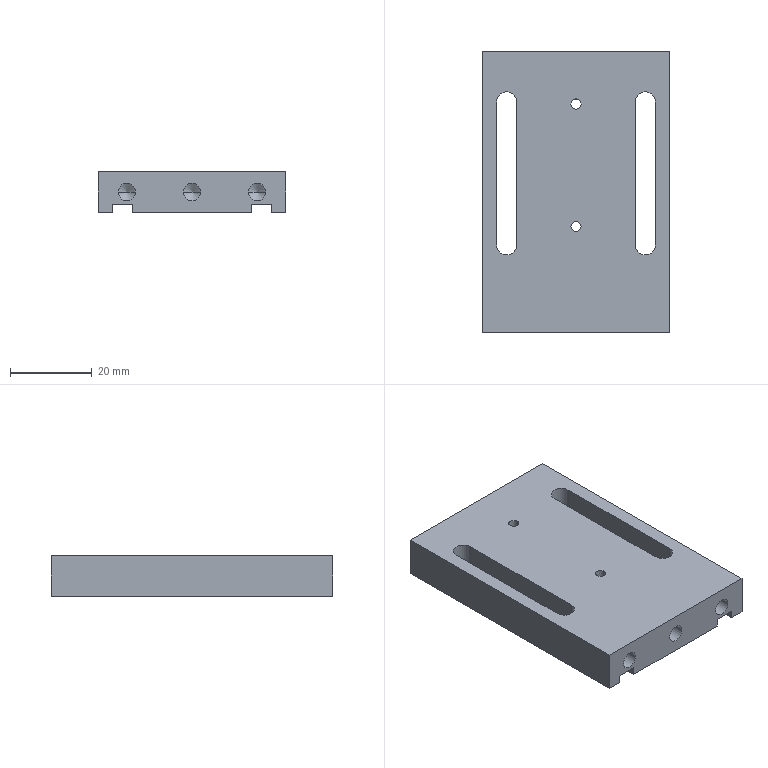Component | SolidWorks | 12-DividingMechanism-1111-1_18-1111-3 | 1 solid | 36 faces | box 46 x 69.1 x 10 mm | volume 26659 mm3 | plane 16 | cylinder 14 | cone 6 | commonest cylinder face diameters 4.2 x6 2.5 x4 5 x4
STEP:
#1=CARTESIAN_POINT('',(0.0523,23.517,60.278));
#2=VERTEX_POINT('',#1);
#3=CARTESIAN_POINT('',(0.2177,23.517,60.278));
#4=VERTEX_POINT('',#3);
#5=CARTESIAN_POINT('',(0.135,23.517,60.278));
#6=DIRECTION('',(-0.,-1.,-0.));
#7=DIRECTION('',(1.,0.,0.));
#8=AXIS2_PLACEMENT_3D('',#5,#6,#7);
#9=CIRCLE('',#8,0.08268);
#10=EDGE_CURVE('',#2,#4,#9,.T.);
#11=ORIENTED_EDGE('',*,*,#10,.F.);
#12=CARTESIAN_POINT('',(0.0523,23.029,60.278));
#13=VERTEX_POINT('',#12);
#14=CARTESIAN_POINT('',(0.0523,23.029,60.278));
#15=DIRECTION('',(-0.,-1.,-0.));
#16=VECTOR('',#15,39.37);
#17=LINE('',#14,#16);
#18=EDGE_CURVE('',#2,#13,#17,.T.);
#19=ORIENTED_EDGE('',*,*,#18,.T.);
#20=CARTESIAN_POINT('',(0.2177,23.029,60.278));
#21=VERTEX_POINT('',#20);
#22=CARTESIAN_POINT('',(0.135,23.029,60.278));
#23=DIRECTION('',(-0.,-1.,-0.));
#24=DIRECTION('',(1.,0.,0.));
#25=AXIS2_PLACEMENT_3D('',#22,#23,#24);
#26=CIRCLE('',#25,0.08268);
#27=EDGE_CURVE('',#13,#21,#26,.T.);
#28=ORIENTED_EDGE('',*,*,#27,.T.);
#29=CARTESIAN_POINT('',(0.2177,23.029,60.278));
#30=DIRECTION('',(-0.,-1.,-0.));
#31=VECTOR('',#30,39.37);
#32=LINE('',#29,#31);
#33=EDGE_CURVE('',#4,#21,#32,.T.);
#34=ORIENTED_EDGE('',*,*,#33,.F.);
#35=EDGE_LOOP('',(#11,#19,#28,#34));
#36=FACE_OUTER_BOUND('',#35,.T.);
#37=CARTESIAN_POINT('',(0.135,23.029,60.278));
#38=DIRECTION('',(-0.,-1.,-0.));
#39=DIRECTION('',(1.,0.,0.));
#40=AXIS2_PLACEMENT_3D('',#37,#38,#39);
#41=CYLINDRICAL_SURFACE('',#40,0.08268);
#42=ADVANCED_FACE('',(#36),#41,.F.);
#43=CARTESIAN_POINT('',(0.135,23.566,60.278));
#44=VERTEX_POINT('',#43);
#45=CARTESIAN_POINT('',(0.2177,23.517,60.278));
#46=DIRECTION('',(0.8572,-0.515,-0.));
#47=VECTOR('',#46,39.37);
#48=LINE('',#45,#47);
#49=EDGE_CURVE('',#44,#4,#48,.T.);
#50=ORIENTED_EDGE('',*,*,#49,.F.);
#51=CARTESIAN_POINT('',(0.0523,23.517,60.278));
#52=DIRECTION('',(-0.8572,-0.515,0.));
#53=VECTOR('',#52,39.37);
#54=LINE('',#51,#53);
#55=EDGE_CURVE('',#44,#2,#54,.T.);
#56=ORIENTED_EDGE('',*,*,#55,.T.);
#57=ORIENTED_EDGE('',*,*,#10,.T.);
#58=EDGE_LOOP('',(#50,#56,#57));
#59=FACE_OUTER_BOUND('',#58,.T.);
#60=CARTESIAN_POINT('',(0.135,23.517,60.278));
#61=DIRECTION('',(-0.,-1.,-0.));
#62=DIRECTION('',(1.,0.,0.));
#63=AXIS2_PLACEMENT_3D('',#60,#61,#62);
#64=CONICAL_SURFACE('',#63,0.08268,1.03);
#65=ADVANCED_FACE('',(#59),#64,.F.);
#66=CARTESIAN_POINT('',(-0.5776,23.517,60.278));
#67=VERTEX_POINT('',#66);
#68=CARTESIAN_POINT('',(-0.4123,23.517,60.278));
#69=VERTEX_POINT('',#68);
#70=CARTESIAN_POINT('',(-0.4949,23.517,60.278));
#71=DIRECTION('',(-0.,-1.,-0.));
#72=DIRECTION('',(1.,0.,0.));
#73=AXIS2_PLACEMENT_3D('',#70,#71,#72);
#74=CIRCLE('',#73,0.08268);
#75=EDGE_CURVE('',#67,#69,#74,.T.);
#76=ORIENTED_EDGE('',*,*,#75,.F.);
#77=CARTESIAN_POINT('',(-0.5776,23.029,60.278));
#78=VERTEX_POINT('',#77);
#79=CARTESIAN_POINT('',(-0.5776,23.029,60.278));
#80=DIRECTION('',(-0.,-1.,-0.));
#81=VECTOR('',#80,39.37);
#82=LINE('',#79,#81);
#83=EDGE_CURVE('',#67,#78,#82,.T.);
#84=ORIENTED_EDGE('',*,*,#83,.T.);
#85=CARTESIAN_POINT('',(-0.4123,23.029,60.278));
#86=VERTEX_POINT('',#85);
#87=CARTESIAN_POINT('',(-0.4949,23.029,60.278));
#88=DIRECTION('',(-0.,-1.,-0.));
#89=DIRECTION('',(1.,0.,0.));
#90=AXIS2_PLACEMENT_3D('',#87,#88,#89);
#91=CIRCLE('',#90,0.08268);
#92=EDGE_CURVE('',#78,#86,#91,.T.);
#93=ORIENTED_EDGE('',*,*,#92,.T.);
#94=CARTESIAN_POINT('',(-0.4123,23.029,60.278));
#95=DIRECTION('',(-0.,-1.,-0.));
#96=VECTOR('',#95,39.37);
#97=LINE('',#94,#96);
#98=EDGE_CURVE('',#69,#86,#97,.T.);
#99=ORIENTED_EDGE('',*,*,#98,.F.);
#100=EDGE_LOOP('',(#76,#84,#93,#99));
#101=FACE_OUTER_BOUND('',#100,.T.);
#102=CARTESIAN_POINT('',(-0.4949,23.029,60.278));
#103=DIRECTION('',(-0.,-1.,-0.));
#104=DIRECTION('',(1.,0.,0.));
#105=AXIS2_PLACEMENT_3D('',#102,#103,#104);
#106=CYLINDRICAL_SURFACE('',#105,0.08268);
#107=ADVANCED_FACE('',(#101),#106,.F.);
#108=CARTESIAN_POINT('',(-0.4949,23.566,60.278));
#109=VERTEX_POINT('',#108);
#110=CARTESIAN_POINT('',(-0.4123,23.517,60.278));
#111=DIRECTION('',(0.8572,-0.515,-0.));
#112=VECTOR('',#111,39.37);
#113=LINE('',#110,#112);
#114=EDGE_CURVE('',#109,#69,#113,.T.);
#115=ORIENTED_EDGE('',*,*,#114,.F.);
#116=CARTESIAN_POINT('',(-0.5776,23.517,60.278));
#117=DIRECTION('',(-0.8572,-0.515,0.));
#118=VECTOR('',#117,39.37);
#119=LINE('',#116,#118);
#120=EDGE_CURVE('',#109,#67,#119,.T.);
#121=ORIENTED_EDGE('',*,*,#120,.T.);
#122=ORIENTED_EDGE('',*,*,#75,.T.);
#123=EDGE_LOOP('',(#115,#121,#122));
#124=FACE_OUTER_BOUND('',#123,.T.);
#125=CARTESIAN_POINT('',(-0.4949,23.517,60.278));
#126=DIRECTION('',(-0.,-1.,-0.));
#127=DIRECTION('',(1.,0.,0.));
#128=AXIS2_PLACEMENT_3D('',#125,#126,#127);
#129=CONICAL_SURFACE('',#128,0.08268,1.03);
#130=ADVANCED_FACE('',(#124),#129,.F.);
#131=CARTESIAN_POINT('',(0.6822,23.517,60.278));
#132=VERTEX_POINT('',#131);
#133=CARTESIAN_POINT('',(0.8476,23.517,60.278));
#134=VERTEX_POINT('',#133);
#135=CARTESIAN_POINT('',(0.7649,23.517,60.278));
#136=DIRECTION('',(-0.,-1.,-0.));
#137=DIRECTION('',(1.,0.,0.));
#138=AXIS2_PLACEMENT_3D('',#135,#136,#137);
#139=CIRCLE('',#138,0.08268);
#140=EDGE_CURVE('',#132,#134,#139,.T.);
#141=ORIENTED_EDGE('',*,*,#140,.F.);
#142=CARTESIAN_POINT('',(0.6822,23.029,60.278));
#143=VERTEX_POINT('',#142);
#144=CARTESIAN_POINT('',(0.6822,23.029,60.278));
#145=DIRECTION('',(-0.,-1.,-0.));
#146=VECTOR('',#145,39.37);
#147=LINE('',#144,#146);
#148=EDGE_CURVE('',#132,#143,#147,.T.);
#149=ORIENTED_EDGE('',*,*,#148,.T.);
#150=CARTESIAN_POINT('',(0.8476,23.029,60.278));
#151=VERTEX_POINT('',#150);
#152=CARTESIAN_POINT('',(0.7649,23.029,60.278));
#153=DIRECTION('',(-0.,-1.,-0.));
#154=DIRECTION('',(1.,0.,0.));
#155=AXIS2_PLACEMENT_3D('',#152,#153,#154);
#156=CIRCLE('',#155,0.08268);
#157=EDGE_CURVE('',#143,#151,#156,.T.);
#158=ORIENTED_EDGE('',*,*,#157,.T.);
#159=CARTESIAN_POINT('',(0.8476,23.029,60.278));
#160=DIRECTION('',(-0.,-1.,-0.));
#161=VECTOR('',#160,39.37);
#162=LINE('',#159,#161);
#163=EDGE_CURVE('',#134,#151,#162,.T.);
#164=ORIENTED_EDGE('',*,*,#163,.F.);
#165=EDGE_LOOP('',(#141,#149,#158,#164));
#166=FACE_OUTER_BOUND('',#165,.T.);
#167=CARTESIAN_POINT('',(0.7649,23.029,60.278));
#168=DIRECTION('',(-0.,-1.,-0.));
#169=DIRECTION('',(1.,0.,0.));
#170=AXIS2_PLACEMENT_3D('',#167,#168,#169);
#171=CYLINDRICAL_SURFACE('',#170,0.08268);
#172=ADVANCED_FACE('',(#166),#171,.F.);
#173=CARTESIAN_POINT('',(0.7649,23.566,60.278));
#174=VERTEX_POINT('',#173);
#175=CARTESIAN_POINT('',(0.8476,23.517,60.278));
#176=DIRECTION('',(0.8572,-0.515,-0.));
#177=VECTOR('',#176,39.37);
#178=LINE('',#175,#177);
#179=EDGE_CURVE('',#174,#134,#178,.T.);
#180=ORIENTED_EDGE('',*,*,#179,.F.);
#181=CARTESIAN_POINT('',(0.6822,23.517,60.278));
#182=DIRECTION('',(-0.8572,-0.515,0.));
#183=VECTOR('',#182,39.37);
#184=LINE('',#181,#183);
#185=EDGE_CURVE('',#174,#132,#184,.T.);
#186=ORIENTED_EDGE('',*,*,#185,.T.);
#187=ORIENTED_EDGE('',*,*,#140,.T.);
#188=EDGE_LOOP('',(#180,#186,#187));
#189=FACE_OUTER_BOUND('',#188,.T.);
#190=CARTESIAN_POINT('',(0.7649,23.517,60.278));
#191=DIRECTION('',(-0.,-1.,-0.));
#192=DIRECTION('',(1.,0.,0.));
#193=AXIS2_PLACEMENT_3D('',#190,#191,#192);
#194=CONICAL_SURFACE('',#193,0.08268,1.03);
#195=ADVANCED_FACE('',(#189),#194,.F.);
#196=CARTESIAN_POINT('',(0.08576,25.237,60.475));
#197=VERTEX_POINT('',#196);
#198=CARTESIAN_POINT('',(0.1842,25.237,60.475));
#199=VERTEX_POINT('',#198);
#200=CARTESIAN_POINT('',(0.135,25.237,60.475));
#201=DIRECTION('',(0.,0.,-1.));
#202=DIRECTION('',(1.,0.,0.));
#203=AXIS2_PLACEMENT_3D('',#200,#201,#202);
#204=CIRCLE('',#203,0.04921);
#205=EDGE_CURVE('',#197,#199,#204,.T.);
#206=ORIENTED_EDGE('',*,*,#205,.F.);
#207=CARTESIAN_POINT('',(0.08576,25.237,60.081));
#208=VERTEX_POINT('',#207);
#209=CARTESIAN_POINT('',(0.08576,25.237,60.081));
#210=DIRECTION('',(0.,0.,-1.));
#211=VECTOR('',#210,39.37);
#212=LINE('',#209,#211);
#213=EDGE_CURVE('',#197,#208,#212,.T.);
#214=ORIENTED_EDGE('',*,*,#213,.T.);
#215=CARTESIAN_POINT('',(0.1842,25.237,60.081));
#216=VERTEX_POINT('',#215);
#217=CARTESIAN_POINT('',(0.135,25.237,60.081));
#218=DIRECTION('',(0.,0.,-1.));
#219=DIRECTION('',(1.,0.,0.));
#220=AXIS2_PLACEMENT_3D('',#217,#218,#219);
#221=CIRCLE('',#220,0.04921);
#222=EDGE_CURVE('',#208,#216,#221,.T.);
#223=ORIENTED_EDGE('',*,*,#222,.T.);
#224=CARTESIAN_POINT('',(0.1842,25.237,60.081));
#225=DIRECTION('',(0.,0.,-1.));
#226=VECTOR('',#225,39.37);
#227=LINE('',#224,#226);
#228=EDGE_CURVE('',#199,#216,#227,.T.);
#229=ORIENTED_EDGE('',*,*,#228,.F.);
#230=EDGE_LOOP('',(#206,#214,#223,#229));
#231=FACE_OUTER_BOUND('',#230,.T.);
#232=CARTESIAN_POINT('',(0.135,25.237,60.081));
#233=DIRECTION('',(0.,0.,-1.));
#234=DIRECTION('',(1.,0.,0.));
#235=AXIS2_PLACEMENT_3D('',#232,#233,#234);
#236=CYLINDRICAL_SURFACE('',#235,0.04921);
#237=ADVANCED_FACE('',(#231),#236,.F.);
#238=CARTESIAN_POINT('',(0.08576,24.056,60.475));
#239=VERTEX_POINT('',#238);
#240=CARTESIAN_POINT('',(0.1842,24.056,60.475));
#241=VERTEX_POINT('',#240);
#242=CARTESIAN_POINT('',(0.135,24.056,60.475));
#243=DIRECTION('',(0.,0.,-1.));
#244=DIRECTION('',(1.,0.,0.));
#245=AXIS2_PLACEMENT_3D('',#242,#243,#244);
#246=CIRCLE('',#245,0.04921);
#247=EDGE_CURVE('',#239,#241,#246,.T.);
#248=ORIENTED_EDGE('',*,*,#247,.F.);
#249=CARTESIAN_POINT('',(0.08576,24.056,60.081));
#250=VERTEX_POINT('',#249);
#251=CARTESIAN_POINT('',(0.08576,24.056,60.081));
#252=DIRECTION('',(0.,0.,-1.));
#253=VECTOR('',#252,39.37);
#254=LINE('',#251,#253);
#255=EDGE_CURVE('',#239,#250,#254,.T.);
#256=ORIENTED_EDGE('',*,*,#255,.T.);
#257=CARTESIAN_POINT('',(0.1842,24.056,60.081));
#258=VERTEX_POINT('',#257);
#259=CARTESIAN_POINT('',(0.135,24.056,60.081));
#260=DIRECTION('',(0.,0.,-1.));
#261=DIRECTION('',(1.,0.,0.));
#262=AXIS2_PLACEMENT_3D('',#259,#260,#261);
#263=CIRCLE('',#262,0.04921);
#264=EDGE_CURVE('',#250,#258,#263,.T.);
#265=ORIENTED_EDGE('',*,*,#264,.T.);
#266=CARTESIAN_POINT('',(0.1842,24.056,60.081));
#267=DIRECTION('',(0.,0.,-1.));
#268=VECTOR('',#267,39.37);
#269=LINE('',#266,#268);
#270=EDGE_CURVE('',#241,#258,#269,.T.);
#271=ORIENTED_EDGE('',*,*,#270,.F.);
#272=EDGE_LOOP('',(#248,#256,#265,#271));
#273=FACE_OUTER_BOUND('',#272,.T.);
#274=CARTESIAN_POINT('',(0.135,24.056,60.081));
#275=DIRECTION('',(0.,0.,-1.));
#276=DIRECTION('',(1.,0.,0.));
#277=AXIS2_PLACEMENT_3D('',#274,#275,#276);
#278=CYLINDRICAL_SURFACE('',#277,0.04921);
#279=ADVANCED_FACE('',(#273),#278,.F.);
#280=CARTESIAN_POINT('',(0.9027,23.029,60.081));
#281=VERTEX_POINT('',#280);
#282=CARTESIAN_POINT('',(1.04,23.029,60.081));
#283=VERTEX_POINT('',#282);
#284=CARTESIAN_POINT('',(-0.7705,23.029,60.081));
#285=DIRECTION('',(1.,-0.,0.));
#286=VECTOR('',#285,39.37);
#287=LINE('',#284,#286);
#288=EDGE_CURVE('',#281,#283,#287,.T.);
#289=ORIENTED_EDGE('',*,*,#288,.F.);
#290=CARTESIAN_POINT('',(0.9027,25.749,60.081));
#291=VERTEX_POINT('',#290);
#292=CARTESIAN_POINT('',(0.9027,25.257,60.081));
#293=DIRECTION('',(0.,1.,0.));
#294=VECTOR('',#293,39.37);
#295=LINE('',#292,#294);
#296=EDGE_CURVE('',#281,#291,#295,.T.);
#297=ORIENTED_EDGE('',*,*,#296,.T.);
#298=CARTESIAN_POINT('',(1.04,25.749,60.081));
#299=VERTEX_POINT('',#298);
#300=CARTESIAN_POINT('',(-0.7705,25.749,60.081));
#301=DIRECTION('',(-1.,0.,0.));
#302=VECTOR('',#301,39.37);
#303=LINE('',#300,#302);
#304=EDGE_CURVE('',#299,#291,#303,.T.);
#305=ORIENTED_EDGE('',*,*,#304,.F.);
#306=CARTESIAN_POINT('',(1.04,23.029,60.081));
#307=DIRECTION('',(0.,1.,0.));
#308=VECTOR('',#307,39.37);
#309=LINE('',#306,#308);
#310=EDGE_CURVE('',#283,#299,#309,.T.);
#311=ORIENTED_EDGE('',*,*,#310,.F.);
#312=EDGE_LOOP('',(#289,#297,#305,#311));
#313=FACE_OUTER_BOUND('',#312,.T.);
#314=CARTESIAN_POINT('',(0.135,24.389,60.081));
#315=DIRECTION('',(-0.,-0.,1.));
#316=DIRECTION('',(-1.,0.,0.));
#317=AXIS2_PLACEMENT_3D('',#314,#315,#316);
#318=PLANE('',#317);
#319=ADVANCED_FACE('',(#313),#318,.F.);
#320=CARTESIAN_POINT('',(-0.6327,25.749,60.081));
#321=VERTEX_POINT('',#320);
#322=CARTESIAN_POINT('',(-0.7705,25.749,60.081));
#323=VERTEX_POINT('',#322);
#324=CARTESIAN_POINT('',(-0.7705,25.749,60.081));
#325=DIRECTION('',(-1.,0.,0.));
#326=VECTOR('',#325,39.37);
#327=LINE('',#324,#326);
#328=EDGE_CURVE('',#321,#323,#327,.T.);
#329=ORIENTED_EDGE('',*,*,#328,.F.);
#330=CARTESIAN_POINT('',(-0.6327,23.029,60.081));
#331=VERTEX_POINT('',#330);
#332=CARTESIAN_POINT('',(-0.6327,25.257,60.081));
#333=DIRECTION('',(-0.,-1.,-0.));
#334=VECTOR('',#333,39.37);
#335=LINE('',#332,#334);
#336=EDGE_CURVE('',#321,#331,#335,.T.);
#337=ORIENTED_EDGE('',*,*,#336,.T.);
#338=CARTESIAN_POINT('',(-0.7705,23.029,60.081));
#339=VERTEX_POINT('',#338);
#340=CARTESIAN_POINT('',(-0.7705,23.029,60.081));
#341=DIRECTION('',(1.,-0.,0.));
#342=VECTOR('',#341,39.37);
#343=LINE('',#340,#342);
#344=EDGE_CURVE('',#339,#331,#343,.T.);
#345=ORIENTED_EDGE('',*,*,#344,.F.);
#346=CARTESIAN_POINT('',(-0.7705,23.029,60.081));
#347=DIRECTION('',(-0.,-1.,-0.));
#348=VECTOR('',#347,39.37);
#349=LINE('',#346,#348);
#350=EDGE_CURVE('',#323,#339,#349,.T.);
#351=ORIENTED_EDGE('',*,*,#350,.F.);
#352=EDGE_LOOP('',(#329,#337,#345,#351));
#353=FACE_OUTER_BOUND('',#352,.T.);
#354=CARTESIAN_POINT('',(0.135,24.389,60.081));
#355=DIRECTION('',(-0.,-0.,1.));
#356=DIRECTION('',(-1.,0.,0.));
#357=AXIS2_PLACEMENT_3D('',#354,#355,#356);
#358=PLANE('',#357);
#359=ADVANCED_FACE('',(#353),#358,.F.);
#360=CARTESIAN_POINT('',(-0.4359,25.257,60.16));
#361=VERTEX_POINT('',#360);
#362=CARTESIAN_POINT('',(-0.6327,25.257,60.16));
#363=VERTEX_POINT('',#362);
#364=CARTESIAN_POINT('',(-0.5343,25.257,60.16));
#365=DIRECTION('',(0.,-0.,1.));
#366=DIRECTION('',(1.,0.,0.));
#367=AXIS2_PLACEMENT_3D('',#364,#365,#366);
#368=CIRCLE('',#367,0.09843);
#369=EDGE_CURVE('',#361,#363,#368,.T.);
#370=ORIENTED_EDGE('',*,*,#369,.F.);
#371=CARTESIAN_POINT('',(-0.4359,25.257,60.475));
#372=VERTEX_POINT('',#371);
#373=CARTESIAN_POINT('',(-0.4359,25.257,60.081));
#374=DIRECTION('',(0.,-0.,1.));
#375=VECTOR('',#374,39.37);
#376=LINE('',#373,#375);
#377=EDGE_CURVE('',#361,#372,#376,.T.);
#378=ORIENTED_EDGE('',*,*,#377,.T.);
#379=CARTESIAN_POINT('',(-0.6327,25.257,60.475));
#380=VERTEX_POINT('',#379);
#381=CARTESIAN_POINT('',(-0.5343,25.257,60.475));
#382=DIRECTION('',(0.,-0.,1.));
#383=DIRECTION('',(-1.,0.,0.));
#384=AXIS2_PLACEMENT_3D('',#381,#382,#383);
#385=CIRCLE('',#384,0.09843);
#386=EDGE_CURVE('',#372,#380,#385,.T.);
#387=ORIENTED_EDGE('',*,*,#386,.T.);
#388=CARTESIAN_POINT('',(-0.6327,25.257,60.081));
#389=DIRECTION('',(0.,-0.,1.));
#390=VECTOR('',#389,39.37);
#391=LINE('',#388,#390);
#392=EDGE_CURVE('',#363,#380,#391,.T.);
#393=ORIENTED_EDGE('',*,*,#392,.F.);
#394=EDGE_LOOP('',(#370,#378,#387,#393));
#395=FACE_OUTER_BOUND('',#394,.T.);
#396=CARTESIAN_POINT('',(-0.5343,25.257,60.081));
#397=DIRECTION('',(0.,-0.,1.));
#398=DIRECTION('',(-1.,0.,0.));
#399=AXIS2_PLACEMENT_3D('',#396,#397,#398);
#400=CYLINDRICAL_SURFACE('',#399,0.09843);
#401=ADVANCED_FACE('',(#395),#400,.F.);
#402=CARTESIAN_POINT('',(-0.6327,23.879,60.16));
#403=VERTEX_POINT('',#402);
#404=CARTESIAN_POINT('',(-0.4359,23.879,60.16));
#405=VERTEX_POINT('',#404);
#406=CARTESIAN_POINT('',(-0.5343,23.879,60.16));
#407=DIRECTION('',(0.,-0.,1.));
#408=DIRECTION('',(1.,0.,0.));
#409=AXIS2_PLACEMENT_3D('',#406,#407,#408);
#410=CIRCLE('',#409,0.09843);
#411=EDGE_CURVE('',#403,#405,#410,.T.);
#412=ORIENTED_EDGE('',*,*,#411,.F.);
#413=CARTESIAN_POINT('',(-0.6327,23.879,60.475));
#414=VERTEX_POINT('',#413);
#415=CARTESIAN_POINT('',(-0.6327,23.879,60.081));
#416=DIRECTION('',(0.,-0.,1.));
#417=VECTOR('',#416,39.37);
#418=LINE('',#415,#417);
#419=EDGE_CURVE('',#403,#414,#418,.T.);
#420=ORIENTED_EDGE('',*,*,#419,.T.);
#421=CARTESIAN_POINT('',(-0.4359,23.879,60.475));
#422=VERTEX_POINT('',#421);
#423=CARTESIAN_POINT('',(-0.5343,23.879,60.475));
#424=DIRECTION('',(0.,-0.,1.));
#425=DIRECTION('',(-1.,0.,0.));
#426=AXIS2_PLACEMENT_3D('',#423,#424,#425);
#427=CIRCLE('',#426,0.09843);
#428=EDGE_CURVE('',#414,#422,#427,.T.);
#429=ORIENTED_EDGE('',*,*,#428,.T.);
#430=CARTESIAN_POINT('',(-0.4359,23.879,60.081));
#431=DIRECTION('',(0.,-0.,1.));
#432=VECTOR('',#431,39.37);
#433=LINE('',#430,#432);
#434=EDGE_CURVE('',#405,#422,#433,.T.);
#435=ORIENTED_EDGE('',*,*,#434,.F.);
#436=EDGE_LOOP('',(#412,#420,#429,#435));
#437=FACE_OUTER_BOUND('',#436,.T.);
#438=CARTESIAN_POINT('',(-0.5343,23.879,60.081));
#439=DIRECTION('',(0.,-0.,1.));
#440=DIRECTION('',(-1.,0.,0.));
#441=AXIS2_PLACEMENT_3D('',#438,#439,#440);
#442=CYLINDRICAL_SURFACE('',#441,0.09843);
#443=ADVANCED_FACE('',(#437),#442,.F.);
#444=ORIENTED_EDGE('',*,*,#304,.T.);
#445=CARTESIAN_POINT('',(0.9027,25.749,60.16));
#446=VERTEX_POINT('',#445);
#447=CARTESIAN_POINT('',(0.9027,25.749,60.16));
#448=DIRECTION('',(0.,0.,-1.));
#449=VECTOR('',#448,39.37);
#450=LINE('',#447,#449);
#451=EDGE_CURVE('',#446,#291,#450,.T.);
#452=ORIENTED_EDGE('',*,*,#451,.F.);
#453=CARTESIAN_POINT('',(0.7058,25.749,60.16));
#454=VERTEX_POINT('',#453);
#455=CARTESIAN_POINT('',(0.7058,25.749,60.16));
#456=DIRECTION('',(1.,-0.,0.));
#457=VECTOR('',#456,39.37);
#458=LINE('',#455,#457);
#459=EDGE_CURVE('',#454,#446,#458,.T.);
#460=ORIENTED_EDGE('',*,*,#459,.F.);
#461=CARTESIAN_POINT('',(0.7058,25.749,60.081));
#462=VERTEX_POINT('',#461);
#463=CARTESIAN_POINT('',(0.7058,25.749,60.16));
#464=DIRECTION('',(0.,0.,-1.));
#465=VECTOR('',#464,39.37);
#466=LINE('',#463,#465);
#467=EDGE_CURVE('',#454,#462,#466,.T.);
#468=ORIENTED_EDGE('',*,*,#467,.T.);
#469=CARTESIAN_POINT('',(-0.4359,25.749,60.081));
#470=VERTEX_POINT('',#469);
#471=CARTESIAN_POINT('',(-0.7705,25.749,60.081));
#472=DIRECTION('',(-1.,0.,0.));
#473=VECTOR('',#472,39.37);
#474=LINE('',#471,#473);
#475=EDGE_CURVE('',#462,#470,#474,.T.);
#476=ORIENTED_EDGE('',*,*,#475,.T.);
#477=CARTESIAN_POINT('',(-0.4359,25.749,60.16));
#478=VERTEX_POINT('',#477);
#479=CARTESIAN_POINT('',(-0.4359,25.749,60.16));
#480=DIRECTION('',(0.,0.,-1.));
#481=VECTOR('',#480,39.37);
#482=LINE('',#479,#481);
#483=EDGE_CURVE('',#478,#470,#482,.T.);
#484=ORIENTED_EDGE('',*,*,#483,.F.);
#485=CARTESIAN_POINT('',(-0.6327,25.749,60.16));
#486=VERTEX_POINT('',#485);
#487=CARTESIAN_POINT('',(-0.4359,25.749,60.16));
#488=DIRECTION('',(1.,-0.,0.));
#489=VECTOR('',#488,39.37);
#490=LINE('',#487,#489);
#491=EDGE_CURVE('',#486,#478,#490,.T.);
#492=ORIENTED_EDGE('',*,*,#491,.F.);
#493=CARTESIAN_POINT('',(-0.6327,25.749,60.16));
#494=DIRECTION('',(0.,0.,-1.));
#495=VECTOR('',#494,39.37);
#496=LINE('',#493,#495);
#497=EDGE_CURVE('',#486,#321,#496,.T.);
#498=ORIENTED_EDGE('',*,*,#497,.T.);
#499=ORIENTED_EDGE('',*,*,#328,.T.);
#500=CARTESIAN_POINT('',(-0.7705,25.749,60.475));
#501=VERTEX_POINT('',#500);
#502=CARTESIAN_POINT('',(-0.7705,25.749,60.475));
#503=DIRECTION('',(0.,0.,-1.));
#504=VECTOR('',#503,39.37);
#505=LINE('',#502,#504);
#506=EDGE_CURVE('',#501,#323,#505,.T.);
#507=ORIENTED_EDGE('',*,*,#506,.F.);
#508=CARTESIAN_POINT('',(1.04,25.749,60.475));
#509=VERTEX_POINT('',#508);
#510=CARTESIAN_POINT('',(-0.7705,25.749,60.475));
#511=DIRECTION('',(-1.,0.,0.));
#512=VECTOR('',#511,39.37);
#513=LINE('',#510,#512);
#514=EDGE_CURVE('',#509,#501,#513,.T.);
#515=ORIENTED_EDGE('',*,*,#514,.F.);
#516=CARTESIAN_POINT('',(1.04,25.749,60.475));
#517=DIRECTION('',(0.,0.,-1.));
#518=VECTOR('',#517,39.37);
#519=LINE('',#516,#518);
#520=EDGE_CURVE('',#509,#299,#519,.T.);
#521=ORIENTED_EDGE('',*,*,#520,.T.);
#522=EDGE_LOOP('',(#444,#452,#460,#468,#476,#484,#492,#498,#499,#507,#515,#521));
#523=FACE_OUTER_BOUND('',#522,.T.);
#524=CARTESIAN_POINT('',(-0.7705,25.749,60.475));
#525=DIRECTION('',(-0.,-1.,-0.));
#526=DIRECTION('',(1.,-0.,0.));
#527=AXIS2_PLACEMENT_3D('',#524,#525,#526);
#528=PLANE('',#527);
#529=ADVANCED_FACE('',(#523),#528,.F.);
#530=ORIENTED_EDGE('',*,*,#350,.T.);
#531=CARTESIAN_POINT('',(-0.7705,23.029,60.475));
#532=VERTEX_POINT('',#531);
#533=CARTESIAN_POINT('',(-0.7705,23.029,60.475));
#534=DIRECTION('',(0.,0.,-1.));
#535=VECTOR('',#534,39.37);
#536=LINE('',#533,#535);
#537=EDGE_CURVE('',#532,#339,#536,.T.);
#538=ORIENTED_EDGE('',*,*,#537,.F.);
#539=CARTESIAN_POINT('',(-0.7705,23.029,60.475));
#540=DIRECTION('',(-0.,-1.,-0.));
#541=VECTOR('',#540,39.37);
#542=LINE('',#539,#541);
#543=EDGE_CURVE('',#501,#532,#542,.T.);
#544=ORIENTED_EDGE('',*,*,#543,.F.);
#545=ORIENTED_EDGE('',*,*,#506,.T.);
#546=EDGE_LOOP('',(#530,#538,#544,#545));
#547=FACE_OUTER_BOUND('',#546,.T.);
#548=CARTESIAN_POINT('',(-0.7705,23.029,60.475));
#549=DIRECTION('',(1.,-0.,0.));
#550=DIRECTION('',(0.,1.,0.));
#551=AXIS2_PLACEMENT_3D('',#548,#549,#550);
#552=PLANE('',#551);
#553=ADVANCED_FACE('',(#547),#552,.F.);
#554=CARTESIAN_POINT('',(0.135,23.029,60.278));
#555=DIRECTION('',(-0.,-1.,-0.));
#556=DIRECTION('',(1.,0.,0.));
#557=AXIS2_PLACEMENT_3D('',#554,#555,#556);
#558=CIRCLE('',#557,0.08268);
#559=EDGE_CURVE('',#21,#13,#558,.T.);
#560=ORIENTED_EDGE('',*,*,#559,.F.);
#561=ORIENTED_EDGE('',*,*,#27,.F.);
#562=EDGE_LOOP('',(#560,#561));
#563=FACE_BOUND('',#562,.T.);
#564=CARTESIAN_POINT('',(-0.4949,23.029,60.278));
#565=DIRECTION('',(-0.,-1.,-0.));
#566=DIRECTION('',(1.,0.,0.));
#567=AXIS2_PLACEMENT_3D('',#564,#565,#566);
#568=CIRCLE('',#567,0.08268);
#569=EDGE_CURVE('',#86,#78,#568,.T.);
#570=ORIENTED_EDGE('',*,*,#569,.F.);
#571=ORIENTED_EDGE('',*,*,#92,.F.);
#572=EDGE_LOOP('',(#570,#571));
#573=FACE_BOUND('',#572,.T.);
#574=CARTESIAN_POINT('',(0.7649,23.029,60.278));
#575=DIRECTION('',(-0.,-1.,-0.));
#576=DIRECTION('',(1.,0.,0.));
#577=AXIS2_PLACEMENT_3D('',#574,#575,#576);
#578=CIRCLE('',#577,0.08268);
#579=EDGE_CURVE('',#151,#143,#578,.T.);
#580=ORIENTED_EDGE('',*,*,#579,.F.);
#581=ORIENTED_EDGE('',*,*,#157,.F.);
#582=EDGE_LOOP('',(#580,#581));
#583=FACE_BOUND('',#582,.T.);
#584=CARTESIAN_POINT('',(0.9027,23.029,60.16));
#585=VERTEX_POINT('',#584);
#586=CARTESIAN_POINT('',(0.7058,23.029,60.16));
#587=VERTEX_POINT('',#586);
#588=CARTESIAN_POINT('',(0.7058,23.029,60.16));
#589=DIRECTION('',(-1.,0.,0.));
#590=VECTOR('',#589,39.37);
#591=LINE('',#588,#590);
#592=EDGE_CURVE('',#585,#587,#591,.T.);
#593=ORIENTED_EDGE('',*,*,#592,.F.);
#594=CARTESIAN_POINT('',(0.9027,23.029,60.16));
#595=DIRECTION('',(0.,0.,-1.));
#596=VECTOR('',#595,39.37);
#597=LINE('',#594,#596);
#598=EDGE_CURVE('',#585,#281,#597,.T.);
#599=ORIENTED_EDGE('',*,*,#598,.T.);
#600=ORIENTED_EDGE('',*,*,#288,.T.);
#601=CARTESIAN_POINT('',(1.04,23.029,60.475));
#602=VERTEX_POINT('',#601);
#603=CARTESIAN_POINT('',(1.04,23.029,60.475));
#604=DIRECTION('',(0.,0.,-1.));
#605=VECTOR('',#604,39.37);
#606=LINE('',#603,#605);
#607=EDGE_CURVE('',#602,#283,#606,.T.);
#608=ORIENTED_EDGE('',*,*,#607,.F.);
#609=CARTESIAN_POINT('',(-0.7705,23.029,60.475));
#610=DIRECTION('',(1.,-0.,0.));
#611=VECTOR('',#610,39.37);
#612=LINE('',#609,#611);
#613=EDGE_CURVE('',#532,#602,#612,.T.);
#614=ORIENTED_EDGE('',*,*,#613,.F.);
#615=ORIENTED_EDGE('',*,*,#537,.T.);
#616=ORIENTED_EDGE('',*,*,#344,.T.);
#617=CARTESIAN_POINT('',(-0.6327,23.029,60.16));
#618=VERTEX_POINT('',#617);
#619=CARTESIAN_POINT('',(-0.6327,23.029,60.16));
#620=DIRECTION('',(0.,0.,-1.));
#621=VECTOR('',#620,39.37);
#622=LINE('',#619,#621);
#623=EDGE_CURVE('',#618,#331,#622,.T.);
#624=ORIENTED_EDGE('',*,*,#623,.F.);
#625=CARTESIAN_POINT('',(-0.4359,23.029,60.16));
#626=VERTEX_POINT('',#625);
#627=CARTESIAN_POINT('',(-0.4359,23.029,60.16));
#628=DIRECTION('',(-1.,0.,0.));
#629=VECTOR('',#628,39.37);
#630=LINE('',#627,#629);
#631=EDGE_CURVE('',#626,#618,#630,.T.);
#632=ORIENTED_EDGE('',*,*,#631,.F.);
#633=CARTESIAN_POINT('',(-0.4359,23.029,60.081));
#634=VERTEX_POINT('',#633);
#635=CARTESIAN_POINT('',(-0.4359,23.029,60.16));
#636=DIRECTION('',(0.,0.,-1.));
#637=VECTOR('',#636,39.37);
#638=LINE('',#635,#637);
#639=EDGE_CURVE('',#626,#634,#638,.T.);
#640=ORIENTED_EDGE('',*,*,#639,.T.);
#641=CARTESIAN_POINT('',(0.7058,23.029,60.081));
#642=VERTEX_POINT('',#641);
#643=CARTESIAN_POINT('',(-0.7705,23.029,60.081));
#644=DIRECTION('',(1.,-0.,0.));
#645=VECTOR('',#644,39.37);
#646=LINE('',#643,#645);
#647=EDGE_CURVE('',#634,#642,#646,.T.);
#648=ORIENTED_EDGE('',*,*,#647,.T.);
#649=CARTESIAN_POINT('',(0.7058,23.029,60.16));
#650=DIRECTION('',(0.,0.,-1.));
#651=VECTOR('',#650,39.37);
#652=LINE('',#649,#651);
#653=EDGE_CURVE('',#587,#642,#652,.T.);
#654=ORIENTED_EDGE('',*,*,#653,.F.);
#655=EDGE_LOOP('',(#593,#599,#600,#608,#614,#615,#616,#624,#632,#640,#648,#654));
#656=FACE_OUTER_BOUND('',#655,.T.);
#657=CARTESIAN_POINT('',(-0.7705,23.029,60.475));
#658=DIRECTION('',(0.,1.,0.));
#659=DIRECTION('',(-1.,0.,0.));
#660=AXIS2_PLACEMENT_3D('',#657,#658,#659);
#661=PLANE('',#660);
#662=ADVANCED_FACE('',(#563,#573,#583,#656),#661,.F.);
#663=ORIENTED_EDGE('',*,*,#310,.T.);
#664=ORIENTED_EDGE('',*,*,#520,.F.);
#665=CARTESIAN_POINT('',(1.04,23.029,60.475));
#666=DIRECTION('',(0.,1.,0.));
#667=VECTOR('',#666,39.37);
#668=LINE('',#665,#667);
#669=EDGE_CURVE('',#602,#509,#668,.T.);
#670=ORIENTED_EDGE('',*,*,#669,.F.);
#671=ORIENTED_EDGE('',*,*,#607,.T.);
#672=EDGE_LOOP('',(#663,#664,#670,#671));
#673=FACE_OUTER_BOUND('',#672,.T.);
#674=CARTESIAN_POINT('',(1.04,23.029,60.475));
#675=DIRECTION('',(-1.,0.,-0.));
#676=DIRECTION('',(-0.,-1.,-0.));
#677=AXIS2_PLACEMENT_3D('',#674,#675,#676);
#678=PLANE('',#677);
#679=ADVANCED_FACE('',(#673),#678,.F.);
#680=CARTESIAN_POINT('',(0.135,25.237,60.475));
#681=DIRECTION('',(0.,0.,-1.));
#682=DIRECTION('',(1.,0.,0.));
#683=AXIS2_PLACEMENT_3D('',#680,#681,#682);
#684=CIRCLE('',#683,0.04921);
#685=EDGE_CURVE('',#199,#197,#684,.T.);
#686=ORIENTED_EDGE('',*,*,#685,.T.);
#687=ORIENTED_EDGE('',*,*,#205,.T.);
#688=EDGE_LOOP('',(#686,#687));
#689=FACE_BOUND('',#688,.T.);
#690=CARTESIAN_POINT('',(0.135,24.056,60.475));
#691=DIRECTION('',(0.,0.,-1.));
#692=DIRECTION('',(1.,0.,0.));
#693=AXIS2_PLACEMENT_3D('',#690,#691,#692);
#694=CIRCLE('',#693,0.04921);
#695=EDGE_CURVE('',#241,#239,#694,.T.);
#696=ORIENTED_EDGE('',*,*,#695,.T.);
#697=ORIENTED_EDGE('',*,*,#247,.T.);
#698=EDGE_LOOP('',(#696,#697));
#699=FACE_BOUND('',#698,.T.);
#700=CARTESIAN_POINT('',(0.9027,25.257,60.475));
#701=VERTEX_POINT('',#700);
#702=CARTESIAN_POINT('',(0.7058,25.257,60.475));
#703=VERTEX_POINT('',#702);
#704=CARTESIAN_POINT('',(0.8043,25.257,60.475));
#705=DIRECTION('',(0.,-0.,1.));
#706=DIRECTION('',(1.,0.,0.));
#707=AXIS2_PLACEMENT_3D('',#704,#705,#706);
#708=CIRCLE('',#707,0.09843);
#709=EDGE_CURVE('',#701,#703,#708,.T.);
#710=ORIENTED_EDGE('',*,*,#709,.F.);
#711=CARTESIAN_POINT('',(0.9027,23.879,60.475));
#712=VERTEX_POINT('',#711);
#713=CARTESIAN_POINT('',(0.9027,25.257,60.475));
#714=DIRECTION('',(0.,1.,0.));
#715=VECTOR('',#714,39.37);
#716=LINE('',#713,#715);
#717=EDGE_CURVE('',#712,#701,#716,.T.);
#718=ORIENTED_EDGE('',*,*,#717,.F.);
#719=CARTESIAN_POINT('',(0.7058,23.879,60.475));
#720=VERTEX_POINT('',#719);
#721=CARTESIAN_POINT('',(0.8043,23.879,60.475));
#722=DIRECTION('',(0.,-0.,1.));
#723=DIRECTION('',(1.,0.,0.));
#724=AXIS2_PLACEMENT_3D('',#721,#722,#723);
#725=CIRCLE('',#724,0.09843);
#726=EDGE_CURVE('',#720,#712,#725,.T.);
#727=ORIENTED_EDGE('',*,*,#726,.F.);
#728=CARTESIAN_POINT('',(0.7058,25.257,60.475));
#729=DIRECTION('',(-0.,-1.,-0.));
#730=VECTOR('',#729,39.37);
#731=LINE('',#728,#730);
#732=EDGE_CURVE('',#703,#720,#731,.T.);
#733=ORIENTED_EDGE('',*,*,#732,.F.);
#734=EDGE_LOOP('',(#710,#718,#727,#733));
#735=FACE_BOUND('',#734,.T.);
#736=ORIENTED_EDGE('',*,*,#386,.F.);
#737=CARTESIAN_POINT('',(-0.4359,25.257,60.475));
#738=DIRECTION('',(0.,1.,0.));
#739=VECTOR('',#738,39.37);
#740=LINE('',#737,#739);
#741=EDGE_CURVE('',#422,#372,#740,.T.);
#742=ORIENTED_EDGE('',*,*,#741,.F.);
#743=ORIENTED_EDGE('',*,*,#428,.F.);
#744=CARTESIAN_POINT('',(-0.6327,25.257,60.475));
#745=DIRECTION('',(-0.,-1.,-0.));
#746=VECTOR('',#745,39.37);
#747=LINE('',#744,#746);
#748=EDGE_CURVE('',#380,#414,#747,.T.);
#749=ORIENTED_EDGE('',*,*,#748,.F.);
#750=EDGE_LOOP('',(#736,#742,#743,#749));
#751=FACE_BOUND('',#750,.T.);
#752=ORIENTED_EDGE('',*,*,#514,.T.);
#753=ORIENTED_EDGE('',*,*,#543,.T.);
#754=ORIENTED_EDGE('',*,*,#613,.T.);
#755=ORIENTED_EDGE('',*,*,#669,.T.);
#756=EDGE_LOOP('',(#752,#753,#754,#755));
#757=FACE_OUTER_BOUND('',#756,.T.);
#758=CARTESIAN_POINT('',(0.135,24.389,60.475));
#759=DIRECTION('',(-0.,-0.,1.));
#760=DIRECTION('',(-1.,0.,0.));
#761=AXIS2_PLACEMENT_3D('',#758,#759,#760);
#762=PLANE('',#761);
#763=ADVANCED_FACE('',(#689,#699,#735,#751,#757),#762,.T.);
#764=CARTESIAN_POINT('',(0.135,25.237,60.081));
#765=DIRECTION('',(0.,0.,-1.));
#766=DIRECTION('',(1.,0.,0.));
#767=AXIS2_PLACEMENT_3D('',#764,#765,#766);
#768=CIRCLE('',#767,0.04921);
#769=EDGE_CURVE('',#216,#208,#768,.T.);
#770=ORIENTED_EDGE('',*,*,#769,.F.);
#771=ORIENTED_EDGE('',*,*,#222,.F.);
#772=EDGE_LOOP('',(#770,#771));
#773=FACE_BOUND('',#772,.T.);
#774=CARTESIAN_POINT('',(0.135,24.056,60.081));
#775=DIRECTION('',(0.,0.,-1.));
#776=DIRECTION('',(1.,0.,0.));
#777=AXIS2_PLACEMENT_3D('',#774,#775,#776);
#778=CIRCLE('',#777,0.04921);
#779=EDGE_CURVE('',#258,#250,#778,.T.);
#780=ORIENTED_EDGE('',*,*,#779,.F.);
#781=ORIENTED_EDGE('',*,*,#264,.F.);
#782=EDGE_LOOP('',(#780,#781));
#783=FACE_BOUND('',#782,.T.);
#784=ORIENTED_EDGE('',*,*,#475,.F.);
#785=CARTESIAN_POINT('',(0.7058,25.257,60.081));
#786=DIRECTION('',(-0.,-1.,-0.));
#787=VECTOR('',#786,39.37);
#788=LINE('',#785,#787);
#789=EDGE_CURVE('',#462,#642,#788,.T.);
#790=ORIENTED_EDGE('',*,*,#789,.T.);
#791=ORIENTED_EDGE('',*,*,#647,.F.);
#792=CARTESIAN_POINT('',(-0.4359,25.257,60.081));
#793=DIRECTION('',(0.,1.,0.));
#794=VECTOR('',#793,39.37);
#795=LINE('',#792,#794);
#796=EDGE_CURVE('',#634,#470,#795,.T.);
#797=ORIENTED_EDGE('',*,*,#796,.T.);
#798=EDGE_LOOP('',(#784,#790,#791,#797));
#799=FACE_OUTER_BOUND('',#798,.T.);
#800=CARTESIAN_POINT('',(0.135,24.389,60.081));
#801=DIRECTION('',(-0.,-0.,1.));
#802=DIRECTION('',(-1.,0.,0.));
#803=AXIS2_PLACEMENT_3D('',#800,#801,#802);
#804=PLANE('',#803);
#805=ADVANCED_FACE('',(#773,#783,#799),#804,.F.);
#806=ORIENTED_EDGE('',*,*,#796,.F.);
#807=ORIENTED_EDGE('',*,*,#639,.F.);
#808=CARTESIAN_POINT('',(-0.4359,23.029,60.16));
#809=DIRECTION('',(-0.,-1.,-0.));
#810=VECTOR('',#809,39.37);
#811=LINE('',#808,#810);
#812=EDGE_CURVE('',#405,#626,#811,.T.);
#813=ORIENTED_EDGE('',*,*,#812,.F.);
#814=ORIENTED_EDGE('',*,*,#434,.T.);
#815=ORIENTED_EDGE('',*,*,#741,.T.);
#816=ORIENTED_EDGE('',*,*,#377,.F.);
#817=CARTESIAN_POINT('',(-0.4359,23.029,60.16));
#818=DIRECTION('',(-0.,-1.,-0.));
#819=VECTOR('',#818,39.37);
#820=LINE('',#817,#819);
#821=EDGE_CURVE('',#478,#361,#820,.T.);
#822=ORIENTED_EDGE('',*,*,#821,.F.);
#823=ORIENTED_EDGE('',*,*,#483,.T.);
#824=EDGE_LOOP('',(#806,#807,#813,#814,#815,#816,#822,#823));
#825=FACE_OUTER_BOUND('',#824,.T.);
#826=CARTESIAN_POINT('',(-0.4359,25.257,60.081));
#827=DIRECTION('',(1.,-0.,0.));
#828=DIRECTION('',(0.,1.,0.));
#829=AXIS2_PLACEMENT_3D('',#826,#827,#828);
#830=PLANE('',#829);
#831=ADVANCED_FACE('',(#825),#830,.F.);
#832=ORIENTED_EDGE('',*,*,#336,.F.);
#833=ORIENTED_EDGE('',*,*,#497,.F.);
#834=CARTESIAN_POINT('',(-0.6327,23.029,60.16));
#835=DIRECTION('',(0.,1.,0.));
#836=VECTOR('',#835,39.37);
#837=LINE('',#834,#836);
#838=EDGE_CURVE('',#363,#486,#837,.T.);
#839=ORIENTED_EDGE('',*,*,#838,.F.);
#840=ORIENTED_EDGE('',*,*,#392,.T.);
#841=ORIENTED_EDGE('',*,*,#748,.T.);
#842=ORIENTED_EDGE('',*,*,#419,.F.);
#843=CARTESIAN_POINT('',(-0.6327,23.029,60.16));
#844=DIRECTION('',(0.,1.,0.));
#845=VECTOR('',#844,39.37);
#846=LINE('',#843,#845);
#847=EDGE_CURVE('',#618,#403,#846,.T.);
#848=ORIENTED_EDGE('',*,*,#847,.F.);
#849=ORIENTED_EDGE('',*,*,#623,.T.);
#850=EDGE_LOOP('',(#832,#833,#839,#840,#841,#842,#848,#849));
#851=FACE_OUTER_BOUND('',#850,.T.);
#852=CARTESIAN_POINT('',(-0.6327,25.257,60.081));
#853=DIRECTION('',(-1.,0.,-0.));
#854=DIRECTION('',(-0.,-1.,-0.));
#855=AXIS2_PLACEMENT_3D('',#852,#853,#854);
#856=PLANE('',#855);
#857=ADVANCED_FACE('',(#851),#856,.F.);
#858=CARTESIAN_POINT('',(0.7058,25.257,60.16));
#859=VERTEX_POINT('',#858);
#860=CARTESIAN_POINT('',(0.7058,25.257,60.081));
#861=DIRECTION('',(0.,-0.,1.));
#862=VECTOR('',#861,39.37);
#863=LINE('',#860,#862);
#864=EDGE_CURVE('',#859,#703,#863,.T.);
#865=ORIENTED_EDGE('',*,*,#864,.F.);
#866=CARTESIAN_POINT('',(0.9027,25.257,60.16));
#867=VERTEX_POINT('',#866);
#868=CARTESIAN_POINT('',(0.8043,25.257,60.16));
#869=DIRECTION('',(0.,0.,-1.));
#870=DIRECTION('',(-1.,0.,0.));
#871=AXIS2_PLACEMENT_3D('',#868,#869,#870);
#872=CIRCLE('',#871,0.09843);
#873=EDGE_CURVE('',#859,#867,#872,.T.);
#874=ORIENTED_EDGE('',*,*,#873,.T.);
#875=CARTESIAN_POINT('',(0.9027,25.257,60.081));
#876=DIRECTION('',(0.,-0.,1.));
#877=VECTOR('',#876,39.37);
#878=LINE('',#875,#877);
#879=EDGE_CURVE('',#867,#701,#878,.T.);
#880=ORIENTED_EDGE('',*,*,#879,.T.);
#881=ORIENTED_EDGE('',*,*,#709,.T.);
#882=EDGE_LOOP('',(#865,#874,#880,#881));
#883=FACE_OUTER_BOUND('',#882,.T.);
#884=CARTESIAN_POINT('',(0.8043,25.257,60.081));
#885=DIRECTION('',(0.,-0.,1.));
#886=DIRECTION('',(-1.,0.,0.));
#887=AXIS2_PLACEMENT_3D('',#884,#885,#886);
#888=CYLINDRICAL_SURFACE('',#887,0.09843);
#889=ADVANCED_FACE('',(#883),#888,.F.);
#890=ORIENTED_EDGE('',*,*,#879,.F.);
#891=CARTESIAN_POINT('',(0.9027,23.029,60.16));
#892=DIRECTION('',(-0.,-1.,-0.));
#893=VECTOR('',#892,39.37);
#894=LINE('',#891,#893);
#895=EDGE_CURVE('',#446,#867,#894,.T.);
#896=ORIENTED_EDGE('',*,*,#895,.F.);
#897=ORIENTED_EDGE('',*,*,#451,.T.);
#898=ORIENTED_EDGE('',*,*,#296,.F.);
#899=ORIENTED_EDGE('',*,*,#598,.F.);
#900=CARTESIAN_POINT('',(0.9027,23.879,60.16));
#901=VERTEX_POINT('',#900);
#902=CARTESIAN_POINT('',(0.9027,23.029,60.16));
#903=DIRECTION('',(-0.,-1.,-0.));
#904=VECTOR('',#903,39.37);
#905=LINE('',#902,#904);
#906=EDGE_CURVE('',#901,#585,#905,.T.);
#907=ORIENTED_EDGE('',*,*,#906,.F.);
#908=CARTESIAN_POINT('',(0.9027,23.879,60.081));
#909=DIRECTION('',(0.,-0.,1.));
#910=VECTOR('',#909,39.37);
#911=LINE('',#908,#910);
#912=EDGE_CURVE('',#901,#712,#911,.T.);
#913=ORIENTED_EDGE('',*,*,#912,.T.);
#914=ORIENTED_EDGE('',*,*,#717,.T.);
#915=EDGE_LOOP('',(#890,#896,#897,#898,#899,#907,#913,#914));
#916=FACE_OUTER_BOUND('',#915,.T.);
#917=CARTESIAN_POINT('',(0.9027,25.257,60.081));
#918=DIRECTION('',(1.,-0.,0.));
#919=DIRECTION('',(0.,1.,0.));
#920=AXIS2_PLACEMENT_3D('',#917,#918,#919);
#921=PLANE('',#920);
#922=ADVANCED_FACE('',(#916),#921,.F.);
#923=ORIENTED_EDGE('',*,*,#912,.F.);
#924=CARTESIAN_POINT('',(0.7058,23.879,60.16));
#925=VERTEX_POINT('',#924);
#926=CARTESIAN_POINT('',(0.8043,23.879,60.16));
#927=DIRECTION('',(0.,0.,-1.));
#928=DIRECTION('',(-1.,0.,0.));
#929=AXIS2_PLACEMENT_3D('',#926,#927,#928);
#930=CIRCLE('',#929,0.09843);
#931=EDGE_CURVE('',#901,#925,#930,.T.);
#932=ORIENTED_EDGE('',*,*,#931,.T.);
#933=CARTESIAN_POINT('',(0.7058,23.879,60.081));
#934=DIRECTION('',(0.,-0.,1.));
#935=VECTOR('',#934,39.37);
#936=LINE('',#933,#935);
#937=EDGE_CURVE('',#925,#720,#936,.T.);
#938=ORIENTED_EDGE('',*,*,#937,.T.);
#939=ORIENTED_EDGE('',*,*,#726,.T.);
#940=EDGE_LOOP('',(#923,#932,#938,#939));
#941=FACE_OUTER_BOUND('',#940,.T.);
#942=CARTESIAN_POINT('',(0.8043,23.879,60.081));
#943=DIRECTION('',(0.,-0.,1.));
#944=DIRECTION('',(-1.,0.,0.));
#945=AXIS2_PLACEMENT_3D('',#942,#943,#944);
#946=CYLINDRICAL_SURFACE('',#945,0.09843);
#947=ADVANCED_FACE('',(#941),#946,.F.);
#948=ORIENTED_EDGE('',*,*,#937,.F.);
#949=CARTESIAN_POINT('',(0.7058,23.029,60.16));
#950=DIRECTION('',(0.,1.,0.));
#951=VECTOR('',#950,39.37);
#952=LINE('',#949,#951);
#953=EDGE_CURVE('',#587,#925,#952,.T.);
#954=ORIENTED_EDGE('',*,*,#953,.F.);
#955=ORIENTED_EDGE('',*,*,#653,.T.);
#956=ORIENTED_EDGE('',*,*,#789,.F.);
#957=ORIENTED_EDGE('',*,*,#467,.F.);
#958=CARTESIAN_POINT('',(0.7058,23.029,60.16));
#959=DIRECTION('',(0.,1.,0.));
#960=VECTOR('',#959,39.37);
#961=LINE('',#958,#960);
#962=EDGE_CURVE('',#859,#454,#961,.T.);
#963=ORIENTED_EDGE('',*,*,#962,.F.);
#964=ORIENTED_EDGE('',*,*,#864,.T.);
#965=ORIENTED_EDGE('',*,*,#732,.T.);
#966=EDGE_LOOP('',(#948,#954,#955,#956,#957,#963,#964,#965));
#967=FACE_OUTER_BOUND('',#966,.T.);
#968=CARTESIAN_POINT('',(0.7058,25.257,60.081));
#969=DIRECTION('',(-1.,0.,-0.));
#970=DIRECTION('',(-0.,-1.,-0.));
#971=AXIS2_PLACEMENT_3D('',#968,#969,#970);
#972=PLANE('',#971);
#973=ADVANCED_FACE('',(#967),#972,.F.);
#974=ORIENTED_EDGE('',*,*,#411,.T.);
#975=ORIENTED_EDGE('',*,*,#812,.T.);
#976=ORIENTED_EDGE('',*,*,#631,.T.);
#977=ORIENTED_EDGE('',*,*,#847,.T.);
#978=EDGE_LOOP('',(#974,#975,#976,#977));
#979=FACE_OUTER_BOUND('',#978,.T.);
#980=CARTESIAN_POINT('',(0.135,24.389,60.16));
#981=DIRECTION('',(0.,0.,-1.));
#982=DIRECTION('',(1.,-0.,0.));
#983=AXIS2_PLACEMENT_3D('',#980,#981,#982);
#984=PLANE('',#983);
#985=ADVANCED_FACE('',(#979),#984,.T.);
#986=ORIENTED_EDGE('',*,*,#369,.T.);
#987=ORIENTED_EDGE('',*,*,#838,.T.);
#988=ORIENTED_EDGE('',*,*,#491,.T.);
#989=ORIENTED_EDGE('',*,*,#821,.T.);
#990=EDGE_LOOP('',(#986,#987,#988,#989));
#991=FACE_OUTER_BOUND('',#990,.T.);
#992=CARTESIAN_POINT('',(0.135,24.389,60.16));
#993=DIRECTION('',(0.,0.,-1.));
#994=DIRECTION('',(1.,-0.,0.));
#995=AXIS2_PLACEMENT_3D('',#992,#993,#994);
#996=PLANE('',#995);
#997=ADVANCED_FACE('',(#991),#996,.T.);
#998=ORIENTED_EDGE('',*,*,#906,.T.);
#999=ORIENTED_EDGE('',*,*,#592,.T.);
#1000=ORIENTED_EDGE('',*,*,#953,.T.);
#1001=ORIENTED_EDGE('',*,*,#931,.F.);
#1002=EDGE_LOOP('',(#998,#999,#1000,#1001));
#1003=FACE_OUTER_BOUND('',#1002,.T.);
#1004=CARTESIAN_POINT('',(0.135,24.389,60.16));
#1005=DIRECTION('',(-0.,-0.,1.));
#1006=DIRECTION('',(-1.,0.,0.));
#1007=AXIS2_PLACEMENT_3D('',#1004,#1005,#1006);
#1008=PLANE('',#1007);
#1009=ADVANCED_FACE('',(#1003),#1008,.F.);
#1010=ORIENTED_EDGE('',*,*,#962,.T.);
#1011=ORIENTED_EDGE('',*,*,#459,.T.);
#1012=ORIENTED_EDGE('',*,*,#895,.T.);
#1013=ORIENTED_EDGE('',*,*,#873,.F.);
#1014=EDGE_LOOP('',(#1010,#1011,#1012,#1013));
#1015=FACE_OUTER_BOUND('',#1014,.T.);
#1016=CARTESIAN_POINT('',(0.135,24.389,60.16));
#1017=DIRECTION('',(-0.,-0.,1.));
#1018=DIRECTION('',(-1.,0.,0.));
#1019=AXIS2_PLACEMENT_3D('',#1016,#1017,#1018);
#1020=PLANE('',#1019);
#1021=ADVANCED_FACE('',(#1015),#1020,.F.);
#1022=ORIENTED_EDGE('',*,*,#255,.F.);
#1023=ORIENTED_EDGE('',*,*,#695,.F.);
#1024=ORIENTED_EDGE('',*,*,#270,.T.);
#1025=ORIENTED_EDGE('',*,*,#779,.T.);
#1026=EDGE_LOOP('',(#1022,#1023,#1024,#1025));
#1027=FACE_OUTER_BOUND('',#1026,.T.);
#1028=CARTESIAN_POINT('',(0.135,24.056,60.081));
#1029=DIRECTION('',(0.,0.,-1.));
#1030=DIRECTION('',(1.,0.,0.));
#1031=AXIS2_PLACEMENT_3D('',#1028,#1029,#1030);
#1032=CYLINDRICAL_SURFACE('',#1031,0.04921);
#1033=ADVANCED_FACE('',(#1027),#1032,.F.);
#1034=ORIENTED_EDGE('',*,*,#213,.F.);
#1035=ORIENTED_EDGE('',*,*,#685,.F.);
#1036=ORIENTED_EDGE('',*,*,#228,.T.);
#1037=ORIENTED_EDGE('',*,*,#769,.T.);
#1038=EDGE_LOOP('',(#1034,#1035,#1036,#1037));
#1039=FACE_OUTER_BOUND('',#1038,.T.);
#1040=CARTESIAN_POINT('',(0.135,25.237,60.081));
#1041=DIRECTION('',(0.,0.,-1.));
#1042=DIRECTION('',(1.,0.,0.));
#1043=AXIS2_PLACEMENT_3D('',#1040,#1041,#1042);
#1044=CYLINDRICAL_SURFACE('',#1043,0.04921);
#1045=ADVANCED_FACE('',(#1039),#1044,.F.);
#1046=ORIENTED_EDGE('',*,*,#185,.F.);
#1047=ORIENTED_EDGE('',*,*,#179,.T.);
#1048=CARTESIAN_POINT('',(0.7649,23.517,60.278));
#1049=DIRECTION('',(-0.,-1.,-0.));
#1050=DIRECTION('',(1.,0.,0.));
#1051=AXIS2_PLACEMENT_3D('',#1048,#1049,#1050);
#1052=CIRCLE('',#1051,0.08268);
#1053=EDGE_CURVE('',#134,#132,#1052,.T.);
#1054=ORIENTED_EDGE('',*,*,#1053,.T.);
#1055=EDGE_LOOP('',(#1046,#1047,#1054));
#1056=FACE_OUTER_BOUND('',#1055,.T.);
#1057=CARTESIAN_POINT('',(0.7649,23.517,60.278));
#1058=DIRECTION('',(-0.,-1.,-0.));
#1059=DIRECTION('',(1.,0.,0.));
#1060=AXIS2_PLACEMENT_3D('',#1057,#1058,#1059);
#1061=CONICAL_SURFACE('',#1060,0.08268,1.03);
#1062=ADVANCED_FACE('',(#1056),#1061,.F.);
#1063=ORIENTED_EDGE('',*,*,#148,.F.);
#1064=ORIENTED_EDGE('',*,*,#1053,.F.);
#1065=ORIENTED_EDGE('',*,*,#163,.T.);
#1066=ORIENTED_EDGE('',*,*,#579,.T.);
#1067=EDGE_LOOP('',(#1063,#1064,#1065,#1066));
#1068=FACE_OUTER_BOUND('',#1067,.T.);
#1069=CARTESIAN_POINT('',(0.7649,23.029,60.278));
#1070=DIRECTION('',(-0.,-1.,-0.));
#1071=DIRECTION('',(1.,0.,0.));
#1072=AXIS2_PLACEMENT_3D('',#1069,#1070,#1071);
#1073=CYLINDRICAL_SURFACE('',#1072,0.08268);
#1074=ADVANCED_FACE('',(#1068),#1073,.F.);
#1075=ORIENTED_EDGE('',*,*,#120,.F.);
#1076=ORIENTED_EDGE('',*,*,#114,.T.);
#1077=CARTESIAN_POINT('',(-0.4949,23.517,60.278));
#1078=DIRECTION('',(-0.,-1.,-0.));
#1079=DIRECTION('',(1.,0.,0.));
#1080=AXIS2_PLACEMENT_3D('',#1077,#1078,#1079);
#1081=CIRCLE('',#1080,0.08268);
#1082=EDGE_CURVE('',#69,#67,#1081,.T.);
#1083=ORIENTED_EDGE('',*,*,#1082,.T.);
#1084=EDGE_LOOP('',(#1075,#1076,#1083));
#1085=FACE_OUTER_BOUND('',#1084,.T.);
#1086=CARTESIAN_POINT('',(-0.4949,23.517,60.278));
#1087=DIRECTION('',(-0.,-1.,-0.));
#1088=DIRECTION('',(1.,0.,0.));
#1089=AXIS2_PLACEMENT_3D('',#1086,#1087,#1088);
#1090=CONICAL_SURFACE('',#1089,0.08268,1.03);
#1091=ADVANCED_FACE('',(#1085),#1090,.F.);
#1092=ORIENTED_EDGE('',*,*,#83,.F.);
#1093=ORIENTED_EDGE('',*,*,#1082,.F.);
#1094=ORIENTED_EDGE('',*,*,#98,.T.);
#1095=ORIENTED_EDGE('',*,*,#569,.T.);
#1096=EDGE_LOOP('',(#1092,#1093,#1094,#1095));
#1097=FACE_OUTER_BOUND('',#1096,.T.);
#1098=CARTESIAN_POINT('',(-0.4949,23.029,60.278));
#1099=DIRECTION('',(-0.,-1.,-0.));
#1100=DIRECTION('',(1.,0.,0.));
#1101=AXIS2_PLACEMENT_3D('',#1098,#1099,#1100);
#1102=CYLINDRICAL_SURFACE('',#1101,0.08268);
#1103=ADVANCED_FACE('',(#1097),#1102,.F.);
#1104=ORIENTED_EDGE('',*,*,#55,.F.);
#1105=ORIENTED_EDGE('',*,*,#49,.T.);
#1106=CARTESIAN_POINT('',(0.135,23.517,60.278));
#1107=DIRECTION('',(-0.,-1.,-0.));
#1108=DIRECTION('',(1.,0.,0.));
#1109=AXIS2_PLACEMENT_3D('',#1106,#1107,#1108);
#1110=CIRCLE('',#1109,0.08268);
#1111=EDGE_CURVE('',#4,#2,#1110,.T.);
#1112=ORIENTED_EDGE('',*,*,#1111,.T.);
#1113=EDGE_LOOP('',(#1104,#1105,#1112));
#1114=FACE_OUTER_BOUND('',#1113,.T.);
#1115=CARTESIAN_POINT('',(0.135,23.517,60.278));
#1116=DIRECTION('',(-0.,-1.,-0.));
#1117=DIRECTION('',(1.,0.,0.));
#1118=AXIS2_PLACEMENT_3D('',#1115,#1116,#1117);
#1119=CONICAL_SURFACE('',#1118,0.08268,1.03);
#1120=ADVANCED_FACE('',(#1114),#1119,.F.);
#1121=ORIENTED_EDGE('',*,*,#18,.F.);
#1122=ORIENTED_EDGE('',*,*,#1111,.F.);
#1123=ORIENTED_EDGE('',*,*,#33,.T.);
#1124=ORIENTED_EDGE('',*,*,#559,.T.);
#1125=EDGE_LOOP('',(#1121,#1122,#1123,#1124));
#1126=FACE_OUTER_BOUND('',#1125,.T.);
#1127=CARTESIAN_POINT('',(0.135,23.029,60.278));
#1128=DIRECTION('',(-0.,-1.,-0.));
#1129=DIRECTION('',(1.,0.,0.));
#1130=AXIS2_PLACEMENT_3D('',#1127,#1128,#1129);
#1131=CYLINDRICAL_SURFACE('',#1130,0.08268);
#1132=ADVANCED_FACE('',(#1126),#1131,.F.);
#1133=CLOSED_SHELL('',(#42,#65,#107,#130,#172,#195,#237,#279,#319,#359,#401,#443,#529,#553,#662,#679,#763,#805,#831,#857,#889,#922,#947,#973,#985,#997,#1009,#1021,#1033,#1045,#1062,#1074,#1091,#1103,#1120,#1132));
#1134=MANIFOLD_SOLID_BREP('',#1133);
#1135=CARTESIAN_POINT('',(0.,0.,0.));
#1136=DIRECTION('',(0.,0.,1.));
#1137=DIRECTION('',(1.,0.,0.));
#1138=AXIS2_PLACEMENT_3D('',#1135,#1136,#1137);
#1139=(LENGTH_UNIT()NAMED_UNIT(*)SI_UNIT($,.METRE.));
#1140=LENGTH_MEASURE_WITH_UNIT(LENGTH_MEASURE(0.0254),#1139);
#1141=DIMENSIONAL_EXPONENTS(1.,0.,0.,0.,0.,0.,0.);
#1142=(CONVERSION_BASED_UNIT('',#1140)LENGTH_UNIT()NAMED_UNIT(#1141));
#1143=UNCERTAINTY_MEASURE_WITH_UNIT(LENGTH_MEASURE(0.00001),#1142,'','');
#1144=(NAMED_UNIT(*)PLANE_ANGLE_UNIT()SI_UNIT($,.RADIAN.));
#1145=(NAMED_UNIT(*)SI_UNIT($,.STERADIAN.)SOLID_ANGLE_UNIT());
#1146=(GEOMETRIC_REPRESENTATION_CONTEXT(3)GLOBAL_UNCERTAINTY_ASSIGNED_CONTEXT((#1143))GLOBAL_UNIT_ASSIGNED_CONTEXT((#1142,#1144,#1145))REPRESENTATION_CONTEXT('',''));
#1147=ADVANCED_BREP_SHAPE_REPRESENTATION('',(#1134,#1138),#1146);
#1148=COLOUR_RGB('',0.7922,0.8196,0.9333);
#1149=FILL_AREA_STYLE_COLOUR('',#1148);
#1150=FILL_AREA_STYLE('',(#1149));
#1151=SURFACE_STYLE_FILL_AREA(#1150);
#1152=SURFACE_SIDE_STYLE('',(#1151));
#1153=SURFACE_STYLE_USAGE(.BOTH.,#1152);
#1154=PRESENTATION_STYLE_ASSIGNMENT((#1153));
#1155=STYLED_ITEM('',(#1154),#1134);
#1156=(LENGTH_UNIT()NAMED_UNIT(*)SI_UNIT($,.METRE.));
#1157=LENGTH_MEASURE_WITH_UNIT(LENGTH_MEASURE(0.0254),#1156);
#1158=DIMENSIONAL_EXPONENTS(1.,0.,0.,0.,0.,0.,0.);
#1159=(CONVERSION_BASED_UNIT('',#1157)LENGTH_UNIT()NAMED_UNIT(#1158));
#1160=UNCERTAINTY_MEASURE_WITH_UNIT(LENGTH_MEASURE(0.00001),#1159,'','');
#1161=(NAMED_UNIT(*)PLANE_ANGLE_UNIT()SI_UNIT($,.RADIAN.));
#1162=(NAMED_UNIT(*)SI_UNIT($,.STERADIAN.)SOLID_ANGLE_UNIT());
#1163=(GEOMETRIC_REPRESENTATION_CONTEXT(3)GLOBAL_UNCERTAINTY_ASSIGNED_CONTEXT((#1160))GLOBAL_UNIT_ASSIGNED_CONTEXT((#1159,#1161,#1162))REPRESENTATION_CONTEXT('',''));
#1164=MECHANICAL_DESIGN_GEOMETRIC_PRESENTATION_REPRESENTATION('',(#1155),#1163);
#1165=PRESENTATION_LAYER_ASSIGNMENT('','',(#1155));